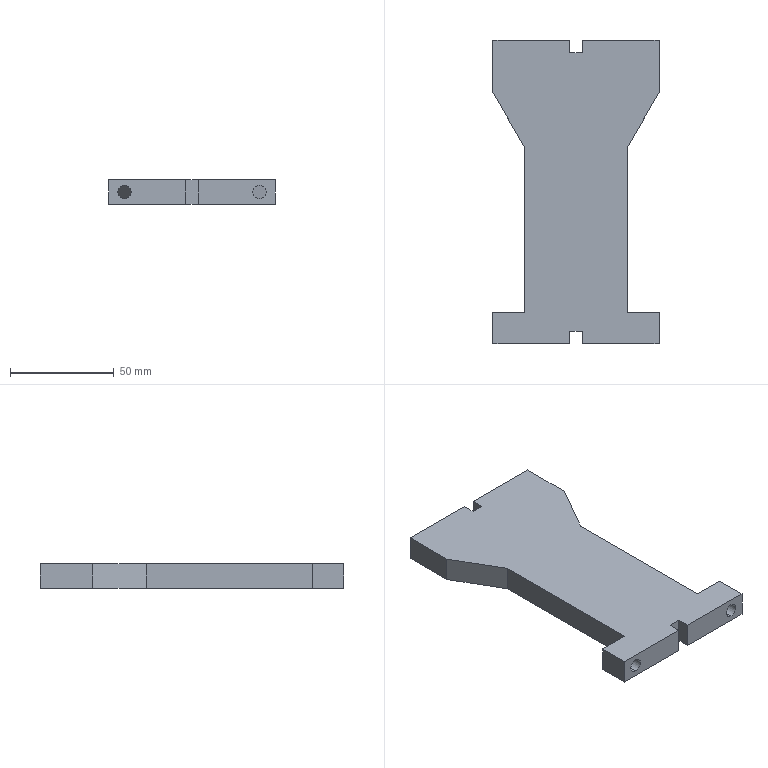Component | SolidWorks | 17268064-1 | 1 solid | 42 faces | box 80 x 146.15 x 12 mm | volume 104257 mm3 | plane 22 | cylinder 12 | cone 8 | commonest cylinder face diameters 4.2 x8 6.5 x4 | material SKD-11 HRC58° Hard Chrome Plated
build123d program:
from build123d import *

# Parameters (mm, degrees)
SKETCH1_W                      = 12
SKETCH1_H                      = 80
BOSS_EXTRUDE1_DEPTH            = 146.15
CUT_EXTRUDE1_DEPTH             = 178.493
F_5_5_5_5_DIAMETER_HOLE1_D     = 6.5
F_5_5_5_5_DIAMETER_HOLE1_DEPTH = 15
M5_TAPPED_HOLE1_D              = 4.2
M5_TAPPED_HOLE1_DEPTH          = 12.4
M5_TAPPED_HOLE1_TIP            = 1.262
SKETCH7_W                      = 6
SKETCH7_H                      = 6
CUT_EXTRUDE2_DEPTH             = 178.493
SKETCH8_W                      = 6
SKETCH8_H                      = 6
CUT_EXTRUDE3_DEPTH             = 178.493


with BuildPart() as part:
    # Sketch1 → Boss-Extrude1 (new body)
    with BuildSketch(Plane.XY):
        with Locations((19, 60)):
            Rectangle(SKETCH1_W, SKETCH1_H)
    extrude(amount=BOSS_EXTRUDE1_DEPTH)

    # Sketch2 → Cut-Extrude1 (cut, through all)
    with BuildSketch(Plane(origin=(25, 0, 0), x_dir=(0, 0, -1), z_dir=(1, 0, 0))):
        Polygon((-131.15, 100), (-131.15, 85), (-51.15, 85), (-25.169, 100), align=None)
        Polygon((-25.169, 20), (-131.15, 20), (-131.15, 35), (-51.15, 35), align=None)
    extrude(amount=-CUT_EXTRUDE1_DEPTH, mode=Mode.SUBTRACT)

    # 5.5 _5.5_ Diameter Hole1
    with Locations(Plane(origin=(0, 0, 131.15), x_dir=(-1, 0, 0), z_dir=(0, 0, -1))):
        with Locations((-19, 92.5), (-19, 27.5)):
            Hole(F_5_5_5_5_DIAMETER_HOLE1_D / 2, depth=F_5_5_5_5_DIAMETER_HOLE1_DEPTH)

    # M5 Tapped Hole1
    with Locations(Plane(origin=(0, 0, 0), x_dir=(-1, 0, 0), z_dir=(0, 0, -1))):
        with Locations((-19, 95), (-19, 25), (-19, 45), (-19, 75)):
            Hole(M5_TAPPED_HOLE1_D / 2, depth=M5_TAPPED_HOLE1_DEPTH)
            with Locations((0, 0, -(M5_TAPPED_HOLE1_DEPTH + M5_TAPPED_HOLE1_TIP / 2))):  # 118° drill point
                Cone(0, M5_TAPPED_HOLE1_D / 2, M5_TAPPED_HOLE1_TIP, mode=Mode.SUBTRACT)

    # Sketch7 → Cut-Extrude2 (cut, through all)
    with BuildSketch(Plane(origin=(25, 0, 0), x_dir=(0, 0, -1), z_dir=(1, 0, 0))):
        with Locations((-3, 60)):
            Rectangle(SKETCH7_W, SKETCH7_H)
    extrude(amount=-CUT_EXTRUDE2_DEPTH, mode=Mode.SUBTRACT)

    # Sketch8 → Cut-Extrude3 (cut, through all)
    with BuildSketch(Plane(origin=(25, 0, 0), x_dir=(0, 0, -1), z_dir=(1, 0, 0))):
        with Locations((-143.15, 60)):
            Rectangle(SKETCH8_W, SKETCH8_H)
    extrude(amount=-CUT_EXTRUDE3_DEPTH, mode=Mode.SUBTRACT)


solid = part.part

# Placed as in the assembly
solid = solid.moved(Location((39.5, -51.579, 0.8507), (90, 0, 90)))